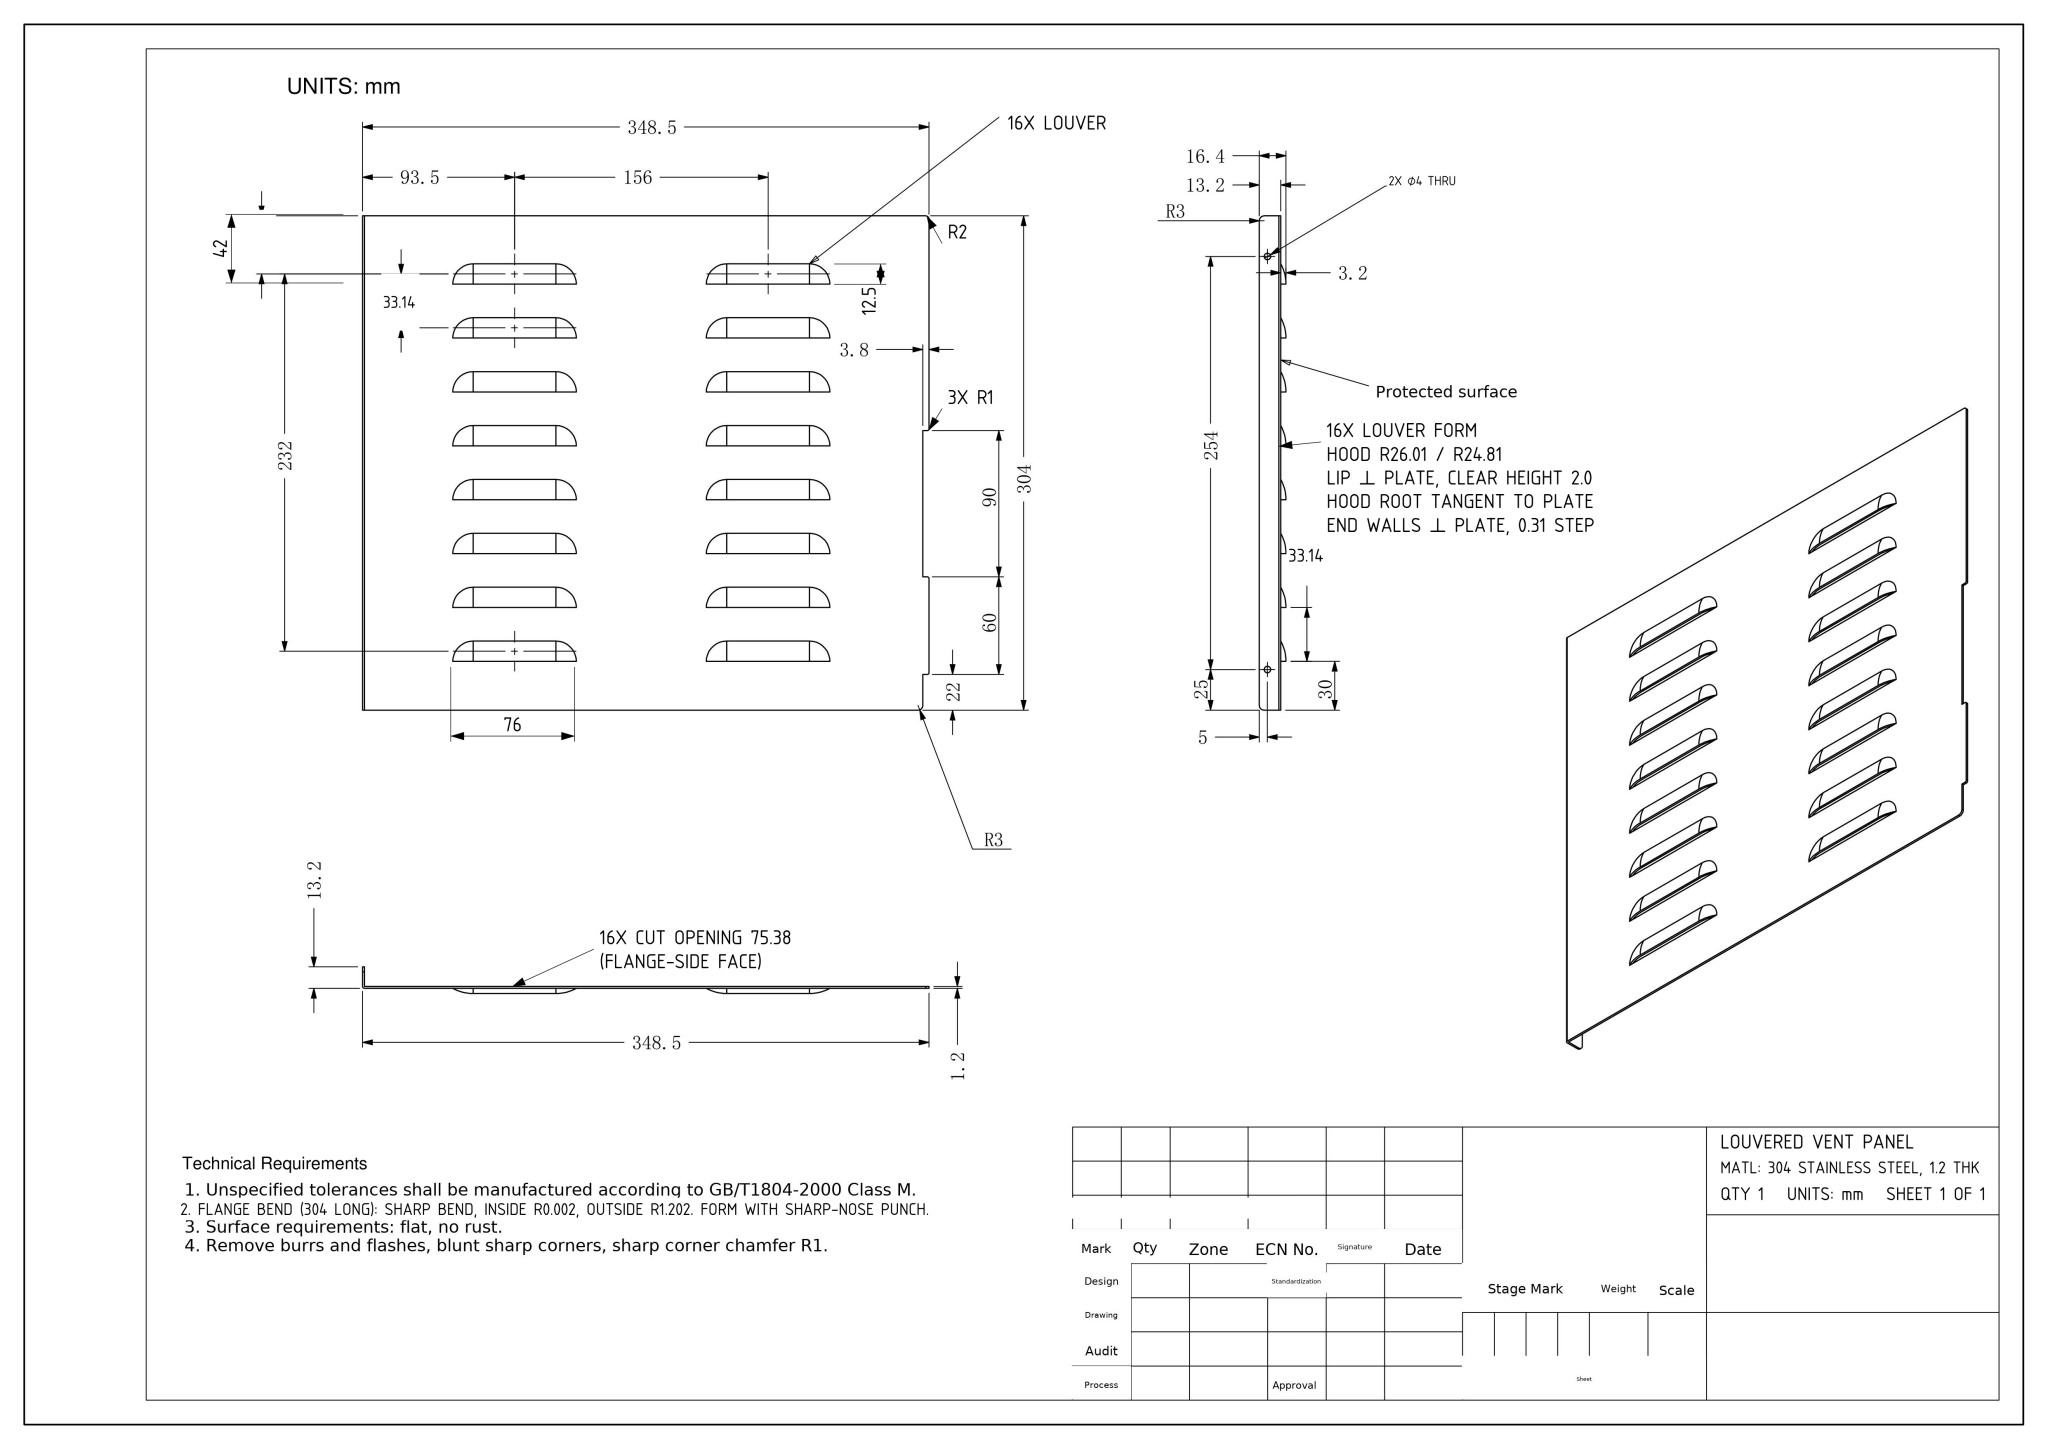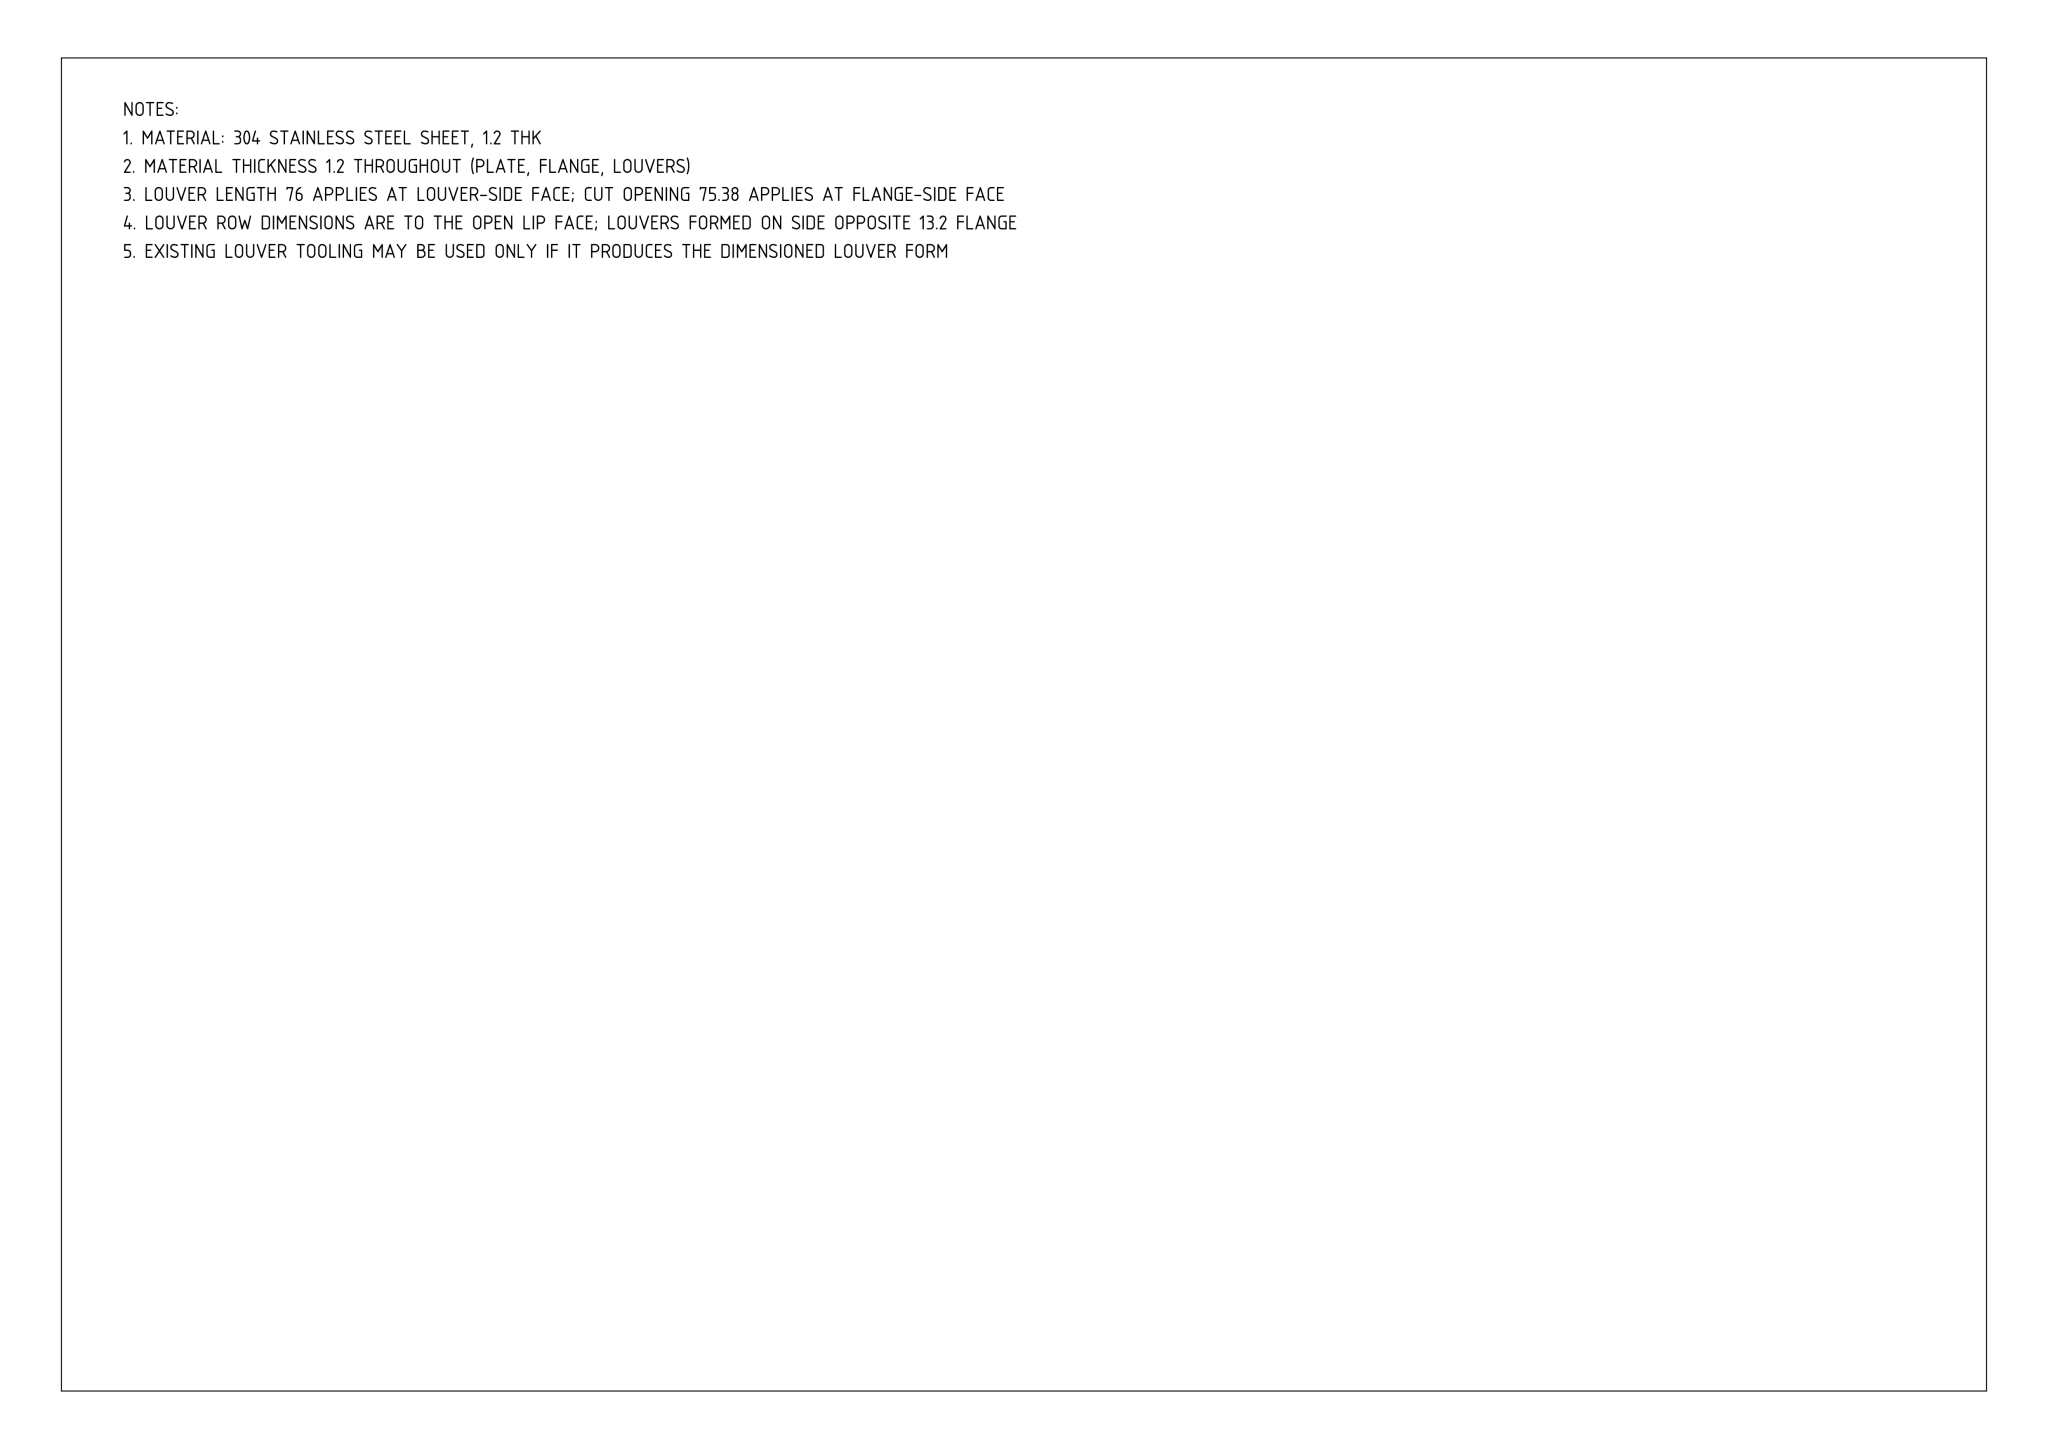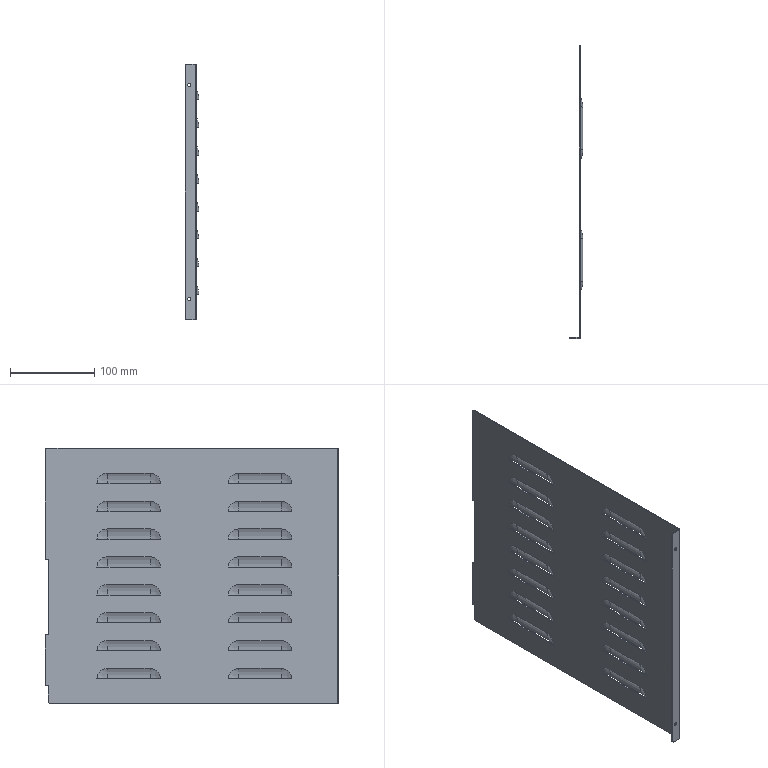Part | NX | mm | 1 solid | 155 faces | box 16.4 x 348.5 x 304 mm | volume 131710 mm3 | sphere 64 | plane 46 | cylinder 45 | commonest cylinder face diameters 52.028 x16 49.628 x16 4 x5 6 x3 2 x3 2.404 x1 0.004 x1